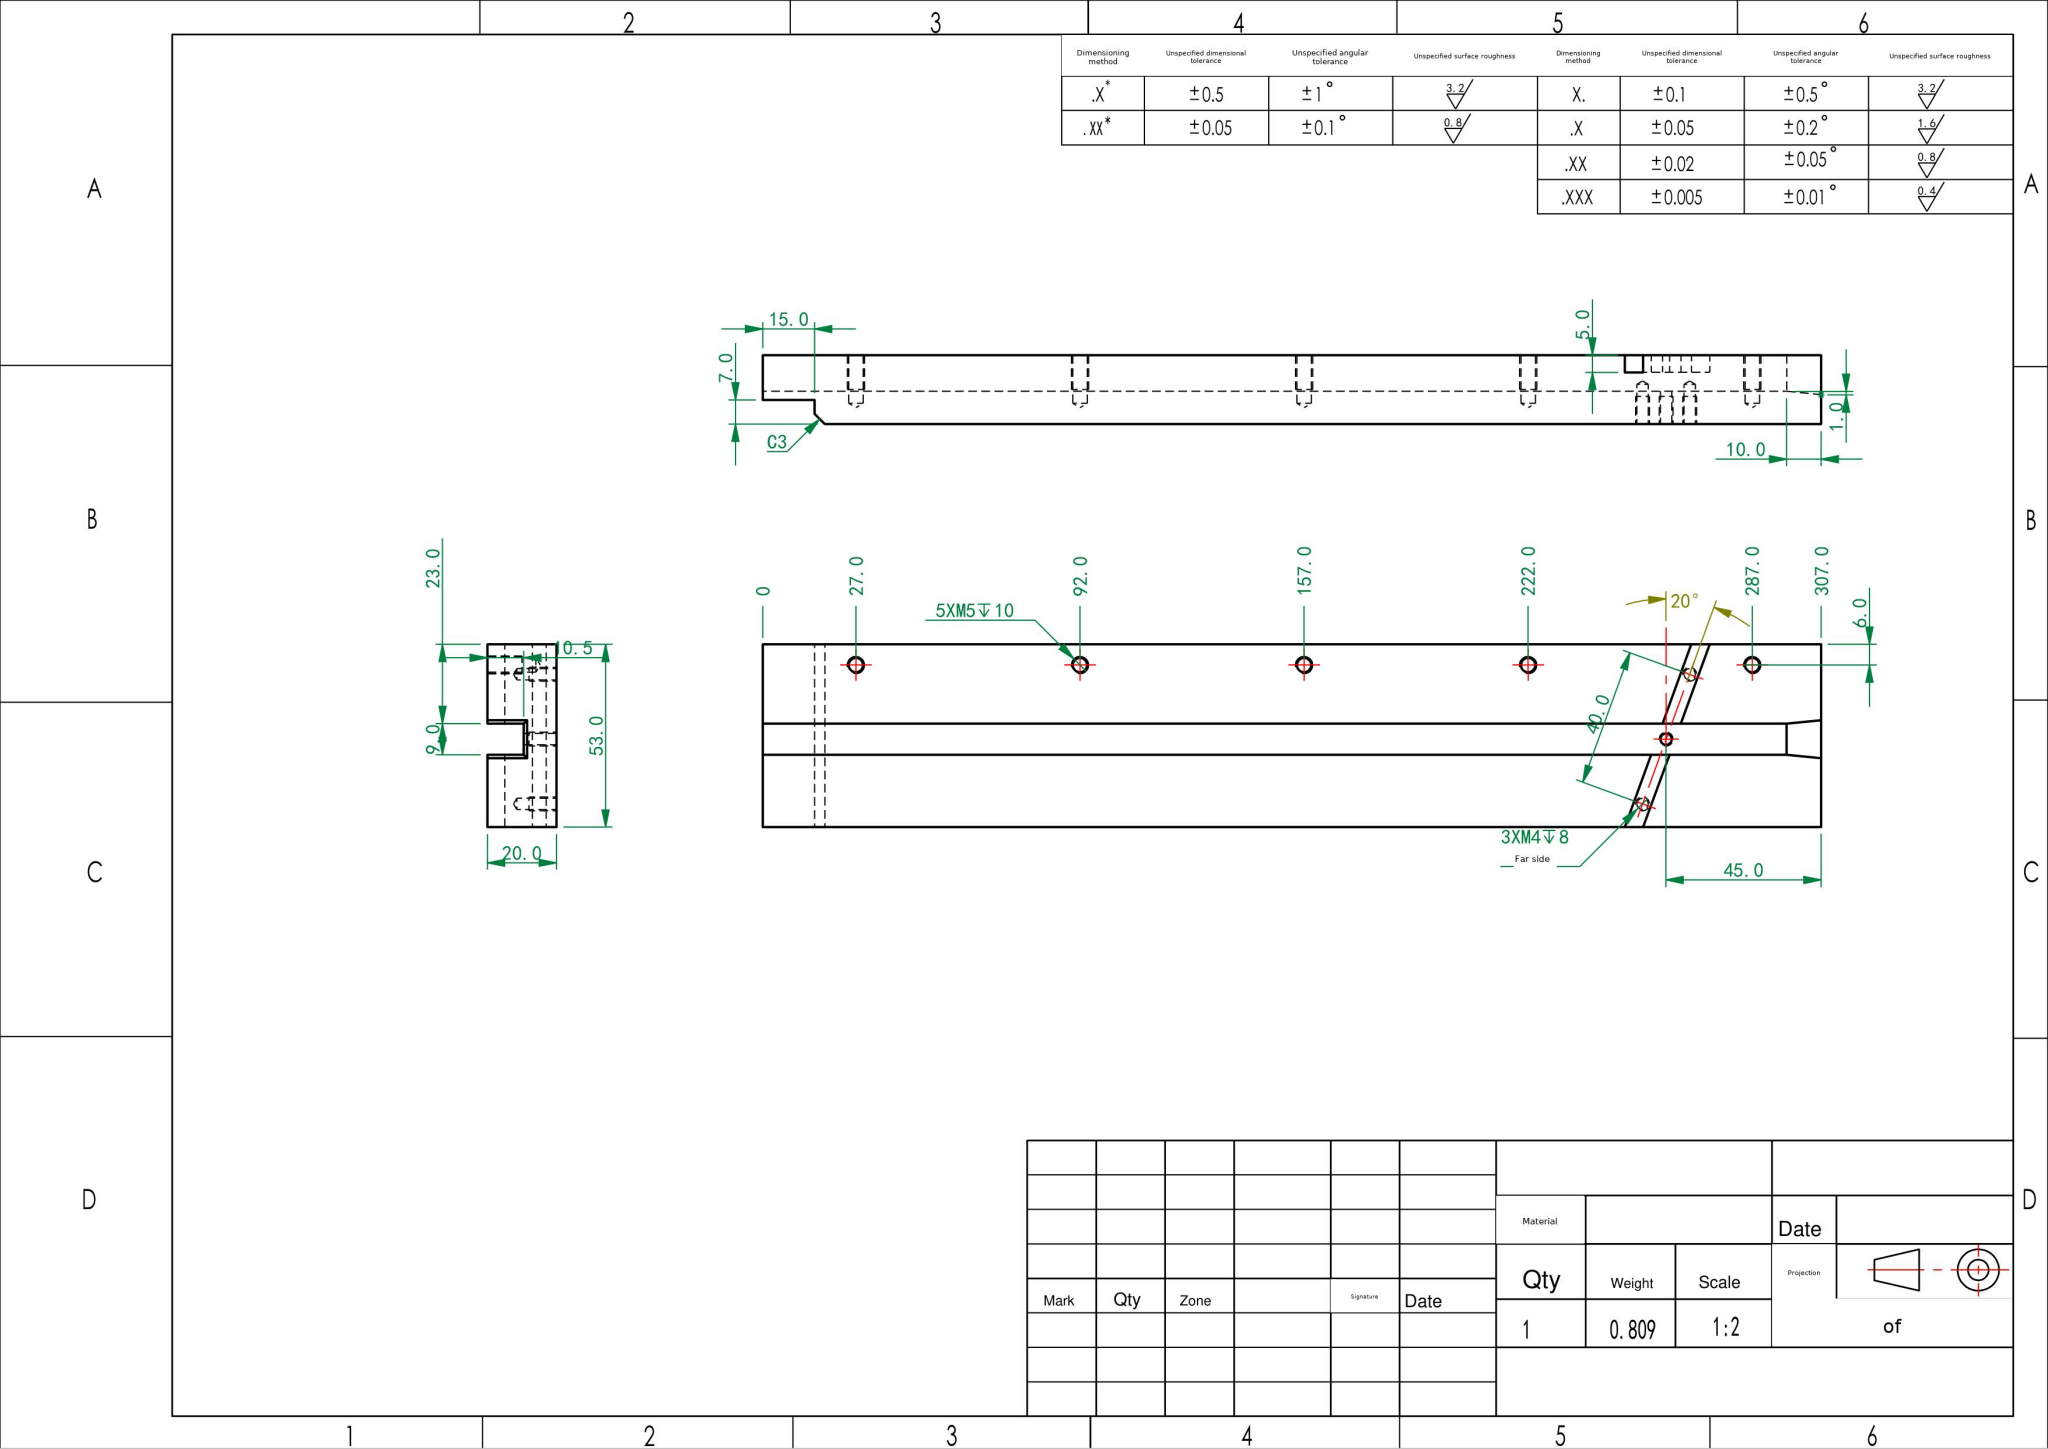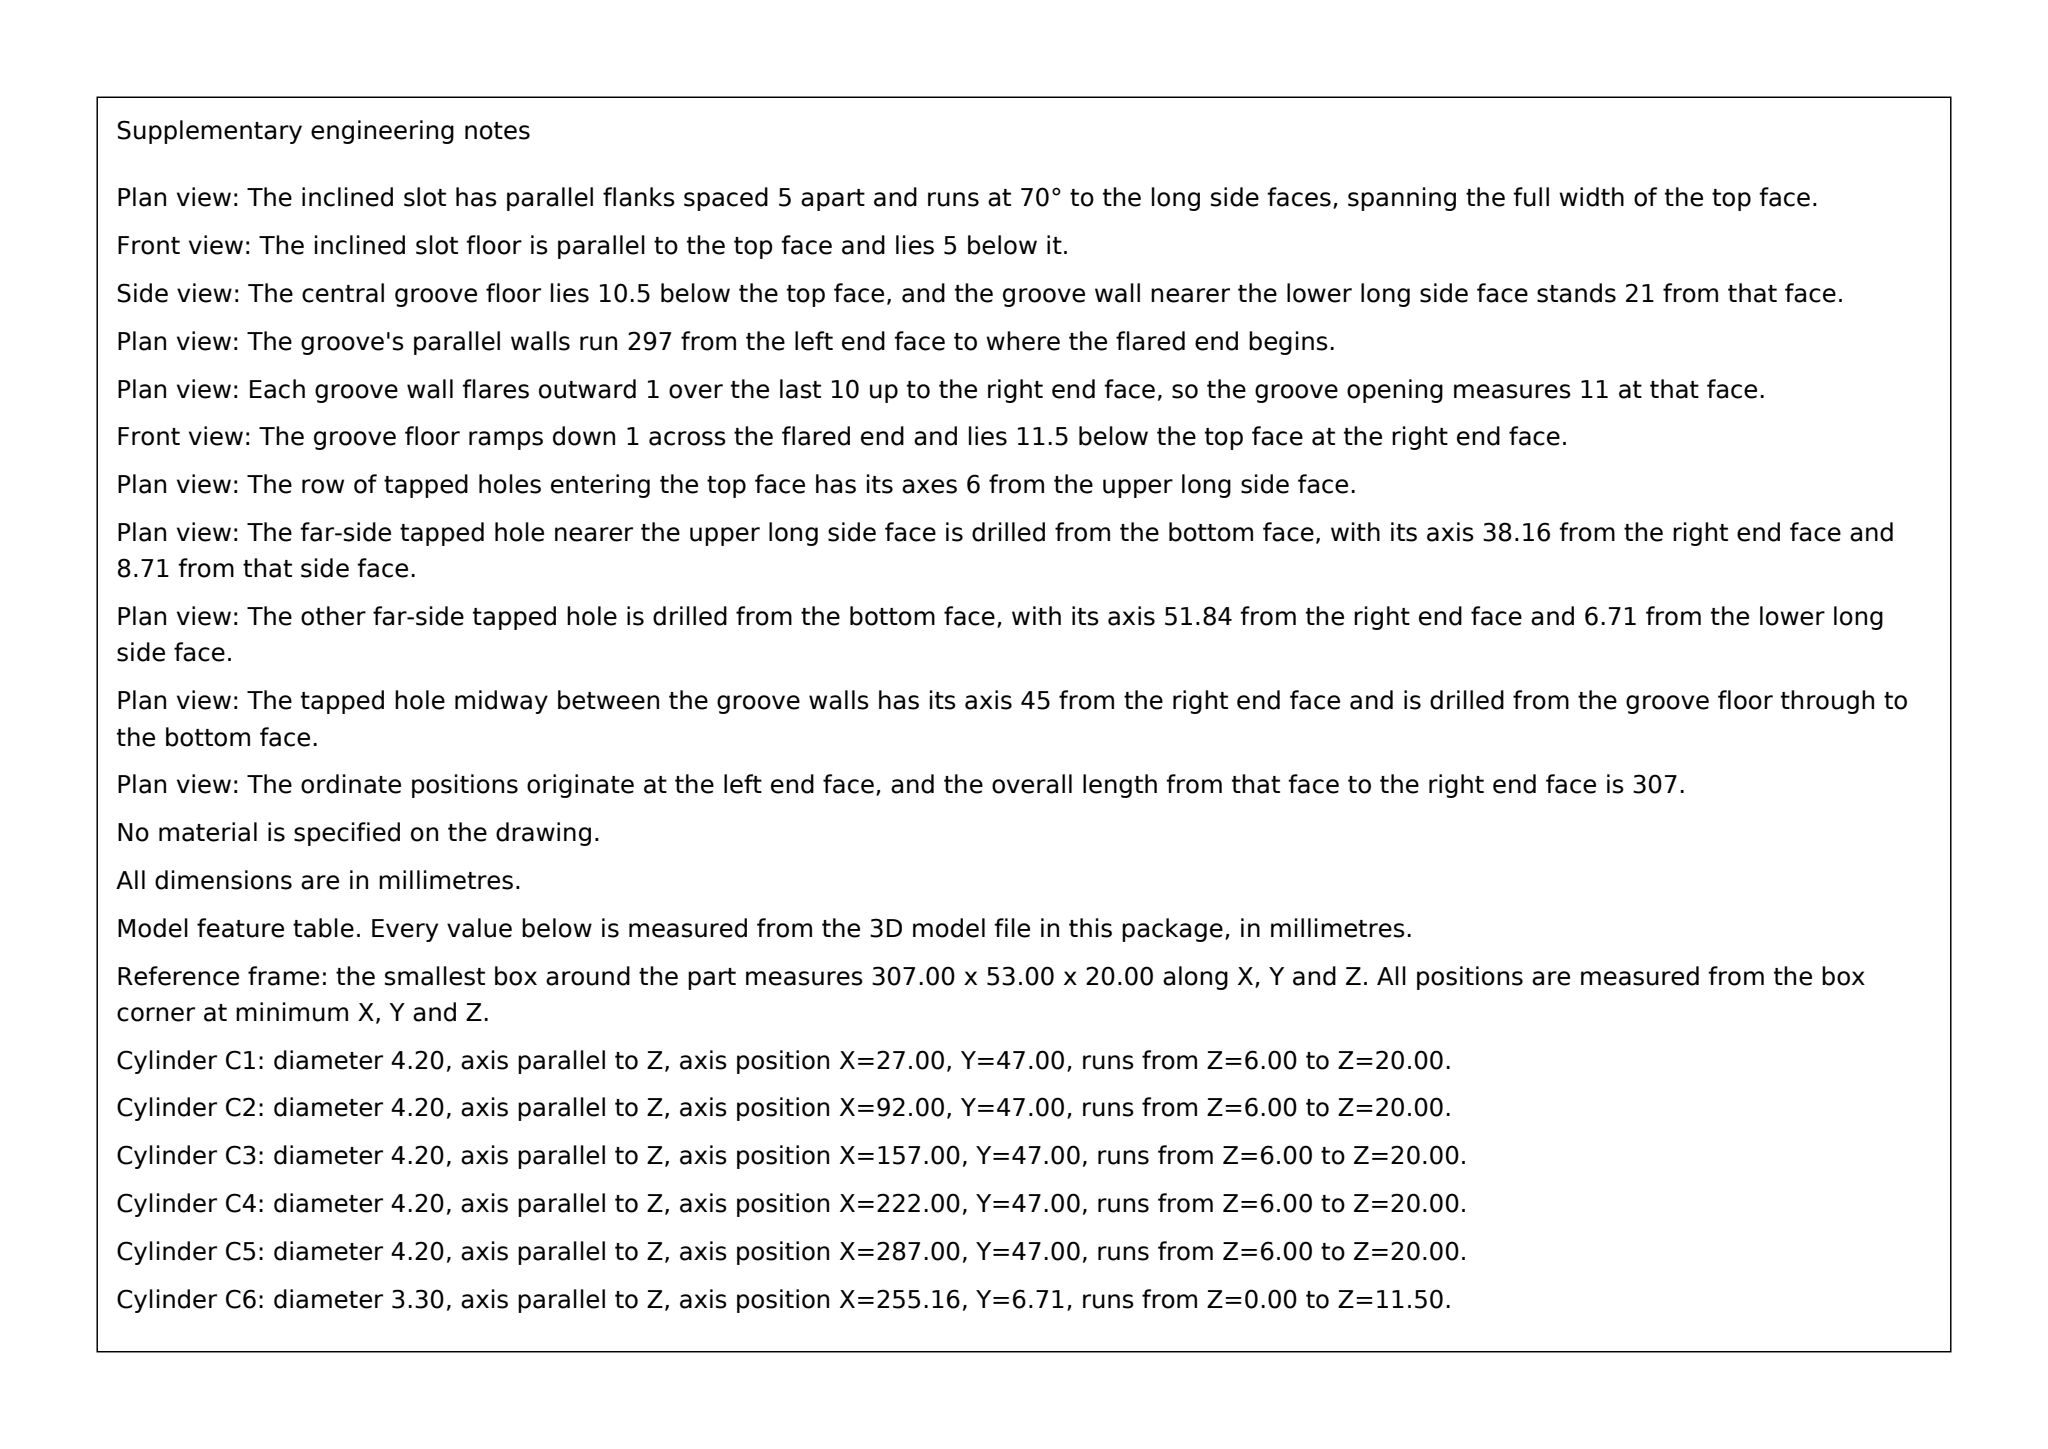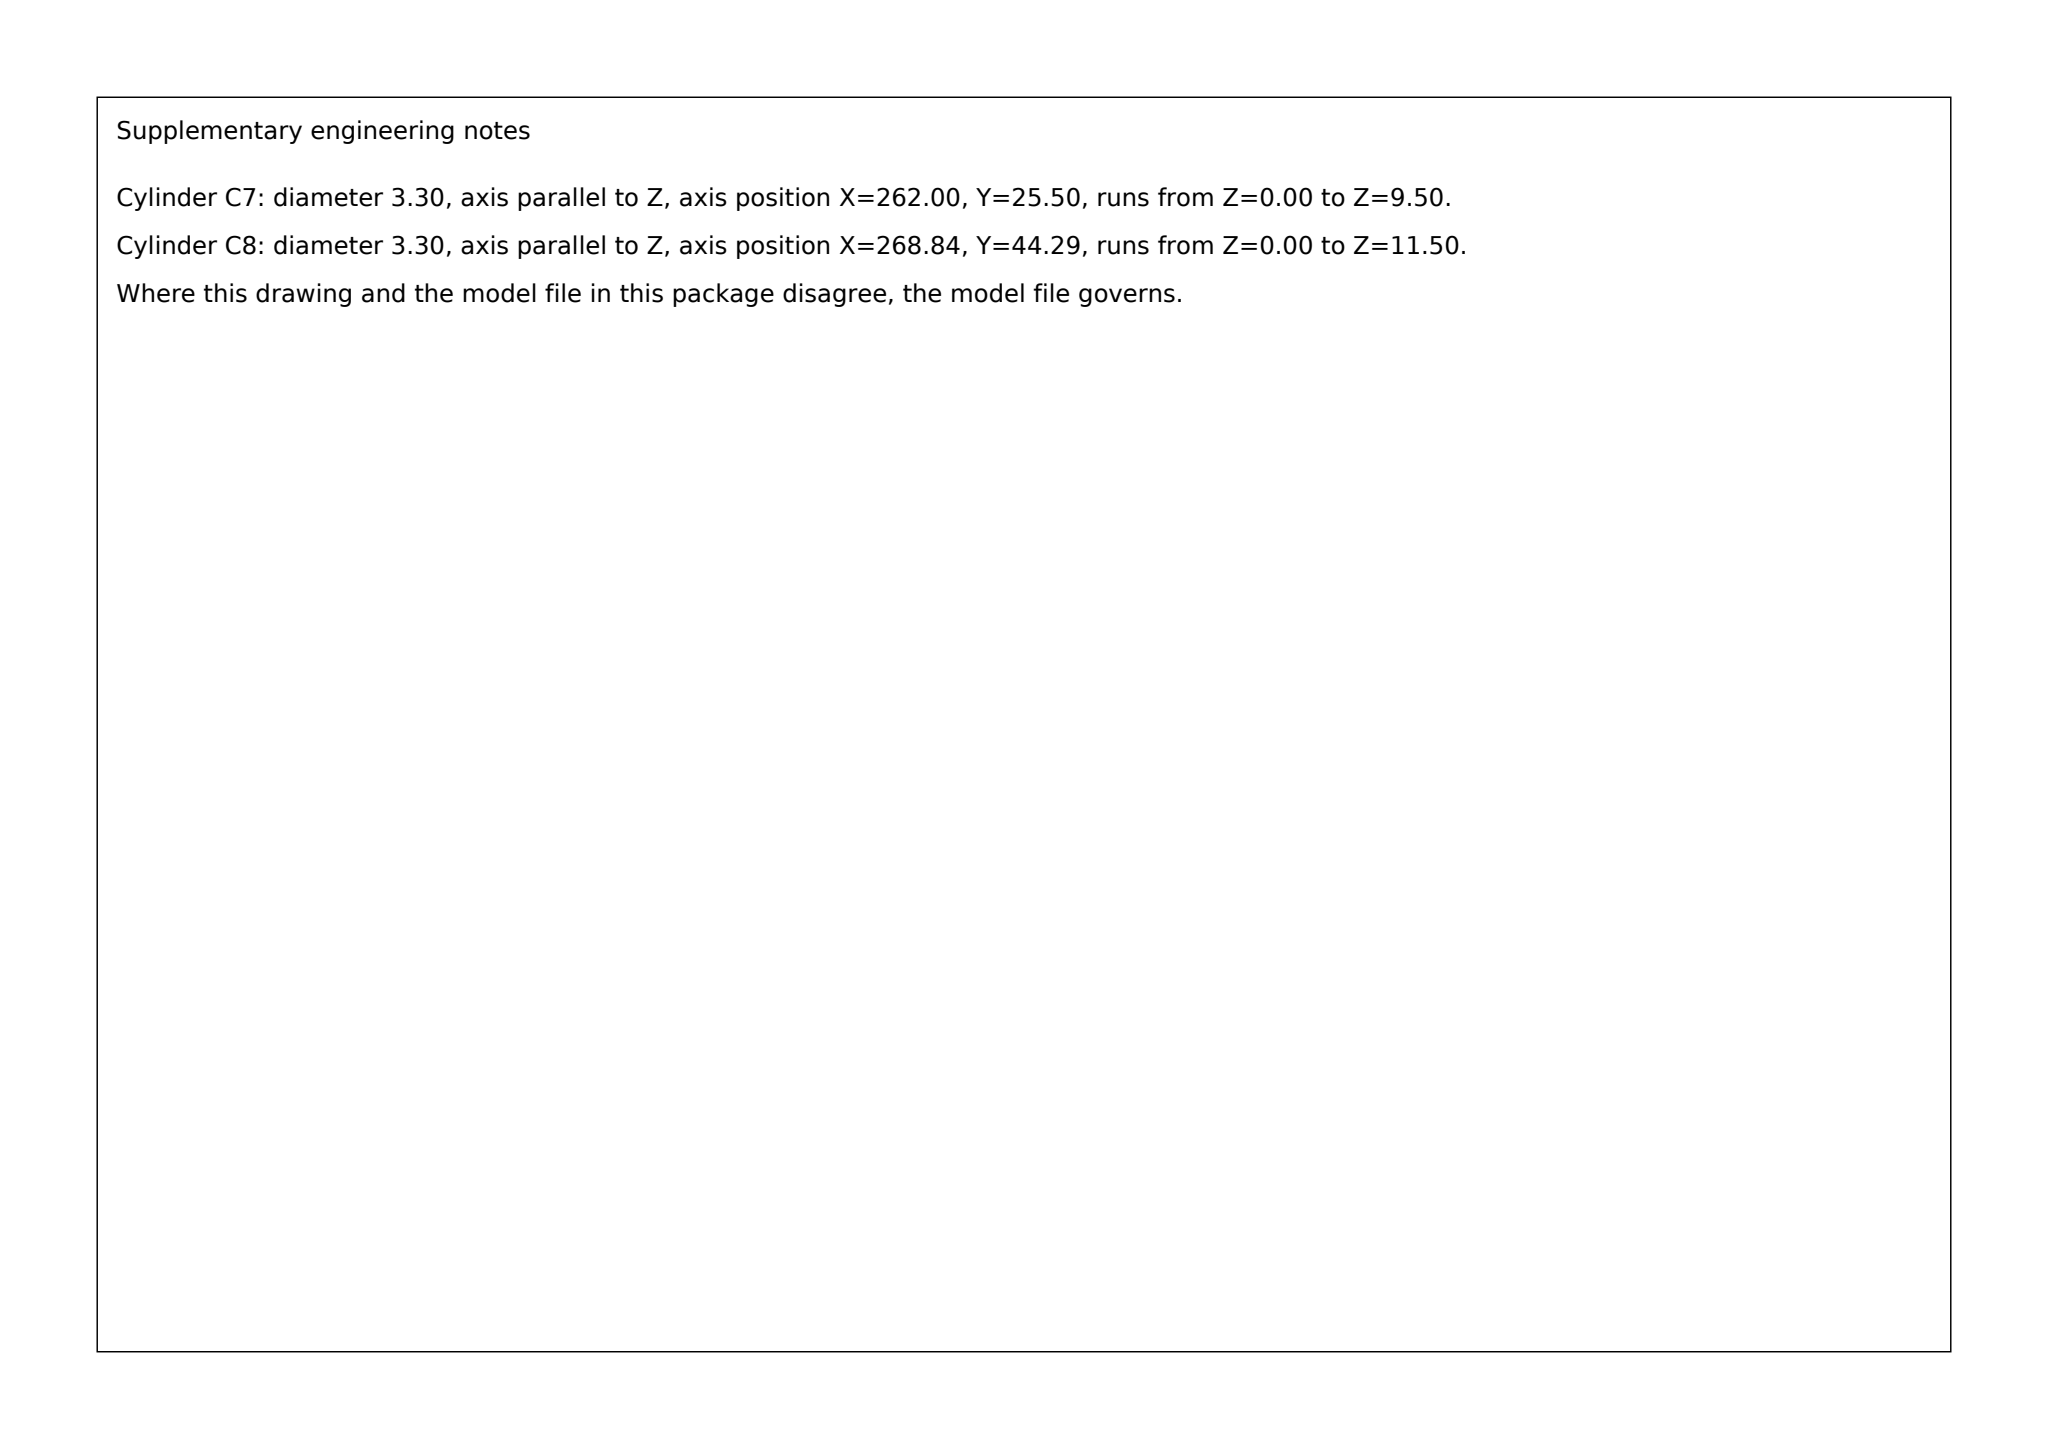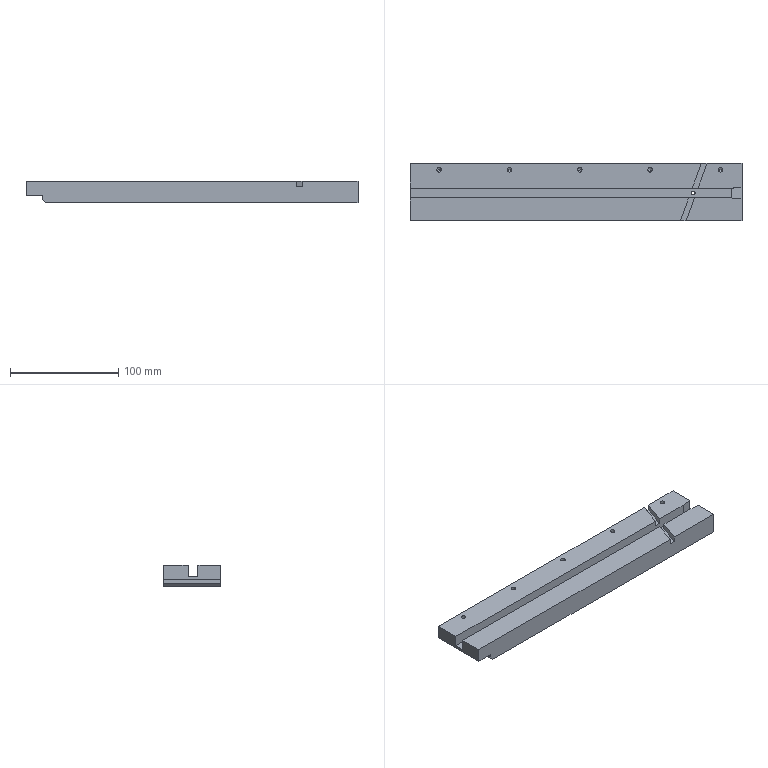Part | SolidWorks | mm | 1 solid | 54 faces | box 307 x 53 x 20 mm | volume 287995 mm3 | plane 24 | cylinder 16 | cone 14 | commonest cylinder face diameters 4.2 x10 3.3 x6
Drawing notes:
9.0 WIDE GROOVE (Y21.0-30.0) RUNS FULL 307.0 LG, OPEN BOTH ENDS | from the solid: y-planes at 21.0 and 30.0 (9.0 apart); bbox X=307.0 with no x-planes bounding groove
build123d program:
from build123d import *

# Parameters (mm, degrees)
SKETCH1_W             = 307
SKETCH1_H             = 55
BOSS_EXTRUDE1_DEPTH   = 20
SKETCH6_W             = 307
SKETCH6_H             = 9
CUT_EXTRUDE1_DEPTH    = 10.5
CHAMFER1_SIZE         = 1
CHAMFER1_SIZE2        = 10
CHAMFER2_SIZE         = 10
CHAMFER2_SIZE2        = 1
LPATTERN1_COUNT       = 5
LPATTERN1_PITCH       = 65
SKETCH15_W            = 15
SKETCH15_H            = 7
CUT_EXTRUDE2_DEPTH    = 55
CHAMFER3_SIZE         = 3
SKETCH16_W            = 307
SKETCH16_H            = 20
CUT_EXTRUDE3_DEPTH    = 2
CUT_EXTRUDE4_DEPTH    = 5
M4_TAPPED_HOLE1_D     = 3.3
M4_TAPPED_HOLE1_DEPTH = 11.5
M4_TAPPED_HOLE1_TIP   = 0.9914
M4_TAPPED_HOLE2_D     = 3.3
M4_TAPPED_HOLE2_DEPTH = 11.5
M4_TAPPED_HOLE2_TIP   = 0.9914


with BuildPart() as part:
    # Sketch1 → Boss-Extrude1 (new body)
    with BuildSketch(Plane.XY):
        Rectangle(SKETCH1_W, SKETCH1_H)
    extrude(amount=BOSS_EXTRUDE1_DEPTH)

    # Sketch6 → Cut-Extrude1 (cut)
    with BuildSketch(Plane.XY.offset(20)):
        Rectangle(SKETCH6_W, SKETCH6_H)
    extrude(amount=-CUT_EXTRUDE1_DEPTH, mode=Mode.SUBTRACT)

    # Chamfer1
    chamfer1_edges = [part.edges().sort_by_distance(p)[0] for p in [
        (153.5, 0, 9.5),
        (153.5, 4.5, 14.75),
    ]]
    chamfer1_side = [part.faces().sort_by_distance(p)[0] for p in [
        (153.5, 0, 0.5852),
    ]]
    chamfer(chamfer1_edges, length=CHAMFER1_SIZE, length2=CHAMFER1_SIZE2, reference=chamfer1_side[0])

    # Chamfer2
    chamfer2_edges = [part.edges().sort_by_distance(p)[0] for p in [
        (153.5, -4.5, 14.25),
    ]]
    chamfer2_side = [part.faces().sort_by_distance(p)[0] for p in [
        (0.2326, -4.5, 14.741),
    ]]
    chamfer(chamfer2_edges, length=CHAMFER2_SIZE, length2=CHAMFER2_SIZE2, reference=chamfer2_side[0])

    # Sketch14 → M5 Tapped Hole1 (revolve, cut)
    with BuildSketch(Plane(origin=(133.5, 21.5, 20), x_dir=(0, -1, 0), z_dir=(1, 0, 0))):
        Polygon((0, 0), (0, 15.262), (2.1, 14), (2.1, 0), align=None)
    m5_tapped_hole1 = revolve(axis=Axis((133.5, 21.5, 26.35), (0, 0, -1)), mode=Mode.SUBTRACT)

    # LPattern1: M5 Tapped Hole1 ×5
    with Locations(*[(-i * LPATTERN1_PITCH, 0, 0) for i in range(1, LPATTERN1_COUNT)]):
        add(m5_tapped_hole1, mode=Mode.SUBTRACT)

    # Sketch15 → Cut-Extrude2 (cut)
    with BuildSketch(Plane.XZ.offset(27.5)):
        with Locations((-146, 3.5)):
            Rectangle(SKETCH15_W, SKETCH15_H)
    extrude(amount=-CUT_EXTRUDE2_DEPTH, mode=Mode.SUBTRACT)

    # Chamfer3
    chamfer3_edges = [part.edges().sort_by_distance(p)[0] for p in [
        (-138.5, 0, 0),
    ]]
    chamfer(chamfer3_edges, length=CHAMFER3_SIZE)

    # Sketch16 → Cut-Extrude3 (cut)
    with BuildSketch(Plane.XZ.offset(27.5)):
        with Locations((0, 10)):
            Rectangle(SKETCH16_W, SKETCH16_H)
    extrude(amount=-CUT_EXTRUDE3_DEPTH, mode=Mode.SUBTRACT)

    # Sketch17 → Cut-Extrude4 (cut)
    with BuildSketch(Plane.XY.offset(20)):
        Polygon((93.325, -34.383), (118.977, 36.094), (123.675, 34.383), (98.023, -36.094), align=None)
    extrude(amount=-CUT_EXTRUDE4_DEPTH, mode=Mode.SUBTRACT)

    # M4 Tapped Hole1
    with Locations(Plane(origin=(108.5, 0, 0), x_dir=(-1, 0, 0), z_dir=(0, 0, -1))):
        with Locations((0, 0)):
            Hole(M4_TAPPED_HOLE1_D / 2, depth=M4_TAPPED_HOLE1_DEPTH)
            with Locations((0, 0, -(M4_TAPPED_HOLE1_DEPTH + M4_TAPPED_HOLE1_TIP / 2))):  # 118° drill point
                Cone(0, M4_TAPPED_HOLE1_D / 2, M4_TAPPED_HOLE1_TIP, mode=Mode.SUBTRACT)

    # M4 Tapped Hole2
    with Locations(Plane(origin=(115.34, 18.794, 0), x_dir=(-1, 0, 0), z_dir=(0, 0, -1))):
        with Locations((0, 0), (13.681, -37.588)):
            Hole(M4_TAPPED_HOLE2_D / 2, depth=M4_TAPPED_HOLE2_DEPTH)
            with Locations((0, 0, -(M4_TAPPED_HOLE2_DEPTH + M4_TAPPED_HOLE2_TIP / 2))):  # 118° drill point
                Cone(0, M4_TAPPED_HOLE2_D / 2, M4_TAPPED_HOLE2_TIP, mode=Mode.SUBTRACT)


solid = part.part